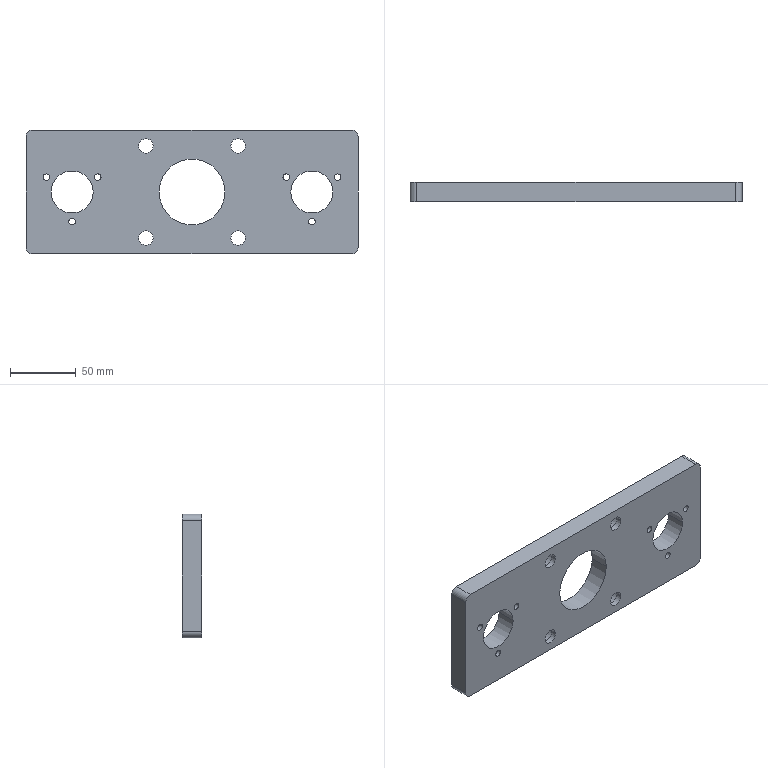Component | SolidWorks | E002GuidePlate-1 | 1 solid | 48 faces | box 252 x 15 x 94 mm | volume 286934 mm3 | cylinder 38 | plane 10 | commonest cylinder face diameters 5 x12 18 x8 11 x8 32 x4 10 x4 50 x2 | material Plain Carbon Steel
build123d program:
from build123d import *

# Parameters (mm, degrees)
SKETCH1_W                                            = 252
SKETCH1_H                                            = 94
BOSS_EXTRUDE1_DEPTH                                  = 7.5
FILLET1_R                                            = 5
SKETCH7_R                                            = 16
CUT_EXTRUDE2_DEPTH                                   = 136.314
CUT_EXTRUDE1_REACH                                   = 137.314
SKETCH6_R                                            = 25
CIRPATTERN1_COUNT                                    = 3
HOLE_SIZE_ACCORDING_TO_THE_TYPE_OF_HEXAG_D           = 11
HOLE_SIZE_ACCORDING_TO_THE_TYPE_OF_HEXAG_CBORE_D     = 18
HOLE_SIZE_ACCORDING_TO_THE_TYPE_OF_HEXAG_CBORE_DEPTH = 11
LPATTERN2_COUNT                                      = 2
LPATTERN2_PITCH                                      = 70
LPATTERN2_COUNT_DIR2                                 = 2
LPATTERN2_PITCH_DIR2                                 = 70


with BuildPart() as part:
    # Sketch1 → Boss-Extrude1 (new, symmetric)
    with BuildSketch(Plane.XY):
        Rectangle(SKETCH1_W, SKETCH1_H)
    extrude(amount=BOSS_EXTRUDE1_DEPTH, both=True)

    # Fillet1
    fillet1_edges = [part.edges().sort_by_distance(p)[0] for p in [
        (126, -47, 0),
        (-126, -47, 0),
        (-126, 47, 0),
        (126, 47, 0),
    ]]
    fillet(fillet1_edges, radius=FILLET1_R)

    # Sketch7 → Cut-Extrude2 (cut, through all)
    with BuildSketch(Plane.XY.offset(7.5)):
        with Locations((-91, 0)):
            Circle(SKETCH7_R)
    cut_extrude2 = extrude(amount=-CUT_EXTRUDE2_DEPTH, mode=Mode.SUBTRACT)

    # Sketch6 → Cut-Extrude1 (cut, up to next)
    with BuildSketch(Plane.XY.offset(7.5), mode=Mode.PRIVATE) as cut_extrude1_sk1:
        Circle(SKETCH6_R)
    cut_extrude1_tool1 = extrude(cut_extrude1_sk1.sketch, amount=-CUT_EXTRUDE1_REACH, mode=Mode.PRIVATE) & part.part
    add(cut_extrude1_tool1.solids().sort_by_distance((0, 0, 7.5))[0], mode=Mode.SUBTRACT)

    # Sketch2 → M6 Tapped Hole1 (revolve, cut)
    with BuildSketch(Plane(origin=(-91, 22.5, 7.5), x_dir=(0, -1, 0), z_dir=(1, 0, 0))):
        Polygon((0, 0), (0, 16.502), (2.5, 15), (2.5, 0), align=None)
    m6_tapped_hole1 = revolve(axis=Axis((-91, 22.5, 13.85), (0, 0, -1)), mode=Mode.SUBTRACT)

    # CirPattern1: M6 Tapped Hole1 ×3 about axis
    cirpattern1_axis = Axis((-91, 0, 0), (0, 0, 1))
    for i in range(1, CIRPATTERN1_COUNT):
        add(m6_tapped_hole1.rotate(cirpattern1_axis, i * 360 / CIRPATTERN1_COUNT), mode=Mode.SUBTRACT)

    # Hole Size according to the type of Hexag (through all)
    with Locations(Plane.XY.offset(7.5)):
        with Locations((-35, 35)):
            hole_size_according_to_the_type_of_hexag = CounterBoreHole(HOLE_SIZE_ACCORDING_TO_THE_TYPE_OF_HEXAG_D / 2, HOLE_SIZE_ACCORDING_TO_THE_TYPE_OF_HEXAG_CBORE_D / 2, HOLE_SIZE_ACCORDING_TO_THE_TYPE_OF_HEXAG_CBORE_DEPTH)

    # LPattern2: Hole Size according to the type of Hexag 2 × 2
    with Locations(*[(i * LPATTERN2_PITCH, -j * LPATTERN2_PITCH_DIR2, 0) for i in range(LPATTERN2_COUNT) for j in range(LPATTERN2_COUNT_DIR2) if (i, j) != (0, 0)]):
        add(hole_size_according_to_the_type_of_hexag, mode=Mode.SUBTRACT)

    # Mirror1: Cut-Extrude2, M6 Tapped Hole1 across plane
    add(cut_extrude2.mirror(Plane(origin=(0, 0, 0), x_dir=(0, 0, 1), z_dir=(1, 0, 0))), mode=Mode.SUBTRACT)
    add(m6_tapped_hole1.mirror(Plane(origin=(0, 0, 0), x_dir=(0, 0, 1), z_dir=(1, 0, 0))), mode=Mode.SUBTRACT)

    # Mirror1 copy 1 sketch → Mirror1 copy 1 (revolve, cut)
    with BuildSketch(Plane(origin=(110.486, -11.25, 7.5), x_dir=(-0.866, 0.5, 0), z_dir=(0.5, 0.866, 0))):
        Polygon((0, 0), (0, -16.502), (2.5, -15), (2.5, 0), align=None)
    revolve(axis=Axis((110.486, -11.25, 13.85), (0, 0, 1)), mode=Mode.SUBTRACT)

    # Mirror1 copy 2 sketch → Mirror1 copy 2 (revolve, cut)
    with BuildSketch(Plane(origin=(71.514, -11.25, 7.5), x_dir=(0.866, 0.5, 0), z_dir=(0.5, -0.866, 0))):
        Polygon((0, 0), (0, -16.502), (2.5, -15), (2.5, 0), align=None)
    revolve(axis=Axis((71.514, -11.25, 13.85), (0, 0, 1)), mode=Mode.SUBTRACT)


solid = part.part

# Placed as in the assembly
solid = solid.moved(Location((0, 205.5, 0), (-90, 0, 0)))